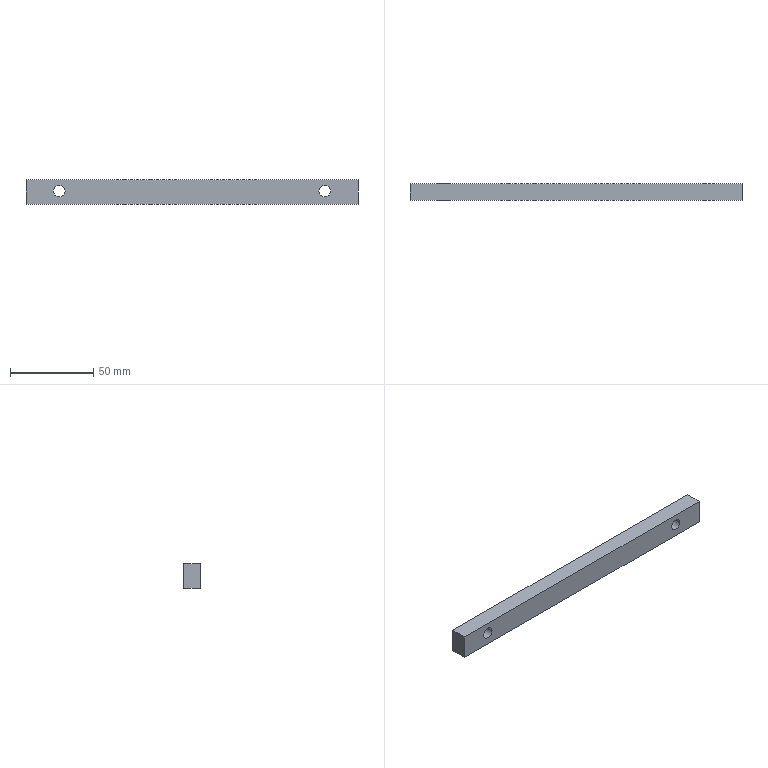Component | SolidWorks | DiscLimitPlateBasePlate-2 | 1 solid | 10 faces | box 200 x 10 x 15 mm | volume 29230 mm3 | plane 6 | cylinder 4 | commonest cylinder face diameters 7 x4
build123d program:
from build123d import *

# Parameters (mm, degrees)
SKETCH1_W      = 200
SKETCH1_H      = 15
SKETCH1_R      = 3.5
EXTRUDE1_DEPTH = 10


with BuildPart() as part:
    # Sketch1 → Extrude1 (new body)
    with BuildSketch(Plane.XY):
        with Locations((71.203, -2.922)):
            Rectangle(SKETCH1_W, SKETCH1_H)
        with Locations((-8.797, -3.422)):
            Circle(SKETCH1_R, mode=Mode.SUBTRACT)
        with Locations((151.203, -3.422)):
            Circle(SKETCH1_R, mode=Mode.SUBTRACT)
    extrude(amount=EXTRUDE1_DEPTH)


solid = part.part

# Placed as in the assembly
solid = solid.moved(Location((-235.987, 430.983, -231.751), (-90, 0, 0)))
STEP:
#1=CARTESIAN_POINT('',(-3.476,17.362,-8.989));
#2=VERTEX_POINT('',#1);
#3=CARTESIAN_POINT('',(-3.2,17.362,-8.989));
#4=VERTEX_POINT('',#3);
#5=CARTESIAN_POINT('',(-3.338,17.362,-8.989));
#6=DIRECTION('',(0.,1.,0.));
#7=DIRECTION('',(1.,0.,0.));
#8=AXIS2_PLACEMENT_3D('',#5,#6,#7);
#9=CIRCLE('',#8,0.1378);
#10=EDGE_CURVE('',#2,#4,#9,.T.);
#11=ORIENTED_EDGE('',*,*,#10,.T.);
#12=CARTESIAN_POINT('',(-3.2,16.968,-8.989));
#13=VERTEX_POINT('',#12);
#14=CARTESIAN_POINT('',(-3.2,17.362,-8.989));
#15=DIRECTION('',(0.,-1.,0.));
#16=VECTOR('',#15,39.37);
#17=LINE('',#14,#16);
#18=EDGE_CURVE('',#4,#13,#17,.T.);
#19=ORIENTED_EDGE('',*,*,#18,.T.);
#20=CARTESIAN_POINT('',(-3.476,16.968,-8.989));
#21=VERTEX_POINT('',#20);
#22=CARTESIAN_POINT('',(-3.338,16.968,-8.989));
#23=DIRECTION('',(0.,1.,0.));
#24=DIRECTION('',(1.,0.,0.));
#25=AXIS2_PLACEMENT_3D('',#22,#23,#24);
#26=CIRCLE('',#25,0.1378);
#27=EDGE_CURVE('',#21,#13,#26,.T.);
#28=ORIENTED_EDGE('',*,*,#27,.F.);
#29=CARTESIAN_POINT('',(-3.476,17.362,-8.989));
#30=DIRECTION('',(0.,-1.,0.));
#31=VECTOR('',#30,39.37);
#32=LINE('',#29,#31);
#33=EDGE_CURVE('',#2,#21,#32,.T.);
#34=ORIENTED_EDGE('',*,*,#33,.F.);
#35=EDGE_LOOP('',(#11,#19,#28,#34));
#36=FACE_OUTER_BOUND('',#35,.T.);
#37=CARTESIAN_POINT('',(-3.338,17.362,-8.989));
#38=DIRECTION('',(0.,-1.,0.));
#39=DIRECTION('',(-1.,0.,0.));
#40=AXIS2_PLACEMENT_3D('',#37,#38,#39);
#41=CYLINDRICAL_SURFACE('',#40,0.1378);
#42=ADVANCED_FACE('',(#36),#41,.F.);
#43=CARTESIAN_POINT('',(-9.775,17.362,-8.989));
#44=VERTEX_POINT('',#43);
#45=CARTESIAN_POINT('',(-9.499,17.362,-8.989));
#46=VERTEX_POINT('',#45);
#47=CARTESIAN_POINT('',(-9.637,17.362,-8.989));
#48=DIRECTION('',(0.,1.,0.));
#49=DIRECTION('',(1.,0.,0.));
#50=AXIS2_PLACEMENT_3D('',#47,#48,#49);
#51=CIRCLE('',#50,0.1378);
#52=EDGE_CURVE('',#44,#46,#51,.T.);
#53=ORIENTED_EDGE('',*,*,#52,.T.);
#54=CARTESIAN_POINT('',(-9.499,16.968,-8.989));
#55=VERTEX_POINT('',#54);
#56=CARTESIAN_POINT('',(-9.499,17.362,-8.989));
#57=DIRECTION('',(0.,-1.,0.));
#58=VECTOR('',#57,39.37);
#59=LINE('',#56,#58);
#60=EDGE_CURVE('',#46,#55,#59,.T.);
#61=ORIENTED_EDGE('',*,*,#60,.T.);
#62=CARTESIAN_POINT('',(-9.775,16.968,-8.989));
#63=VERTEX_POINT('',#62);
#64=CARTESIAN_POINT('',(-9.637,16.968,-8.989));
#65=DIRECTION('',(0.,1.,0.));
#66=DIRECTION('',(1.,0.,0.));
#67=AXIS2_PLACEMENT_3D('',#64,#65,#66);
#68=CIRCLE('',#67,0.1378);
#69=EDGE_CURVE('',#63,#55,#68,.T.);
#70=ORIENTED_EDGE('',*,*,#69,.F.);
#71=CARTESIAN_POINT('',(-9.775,17.362,-8.989));
#72=DIRECTION('',(0.,-1.,0.));
#73=VECTOR('',#72,39.37);
#74=LINE('',#71,#73);
#75=EDGE_CURVE('',#44,#63,#74,.T.);
#76=ORIENTED_EDGE('',*,*,#75,.F.);
#77=EDGE_LOOP('',(#53,#61,#70,#76));
#78=FACE_OUTER_BOUND('',#77,.T.);
#79=CARTESIAN_POINT('',(-9.637,17.362,-8.989));
#80=DIRECTION('',(0.,-1.,0.));
#81=DIRECTION('',(-1.,0.,0.));
#82=AXIS2_PLACEMENT_3D('',#79,#80,#81);
#83=CYLINDRICAL_SURFACE('',#82,0.1378);
#84=ADVANCED_FACE('',(#78),#83,.F.);
#85=ORIENTED_EDGE('',*,*,#52,.F.);
#86=CARTESIAN_POINT('',(-9.637,17.362,-8.989));
#87=DIRECTION('',(0.,1.,0.));
#88=DIRECTION('',(1.,0.,0.));
#89=AXIS2_PLACEMENT_3D('',#86,#87,#88);
#90=CIRCLE('',#89,0.1378);
#91=EDGE_CURVE('',#46,#44,#90,.T.);
#92=ORIENTED_EDGE('',*,*,#91,.F.);
#93=EDGE_LOOP('',(#85,#92));
#94=FACE_BOUND('',#93,.T.);
#95=CARTESIAN_POINT('',(-10.425,17.362,-9.304));
#96=VERTEX_POINT('',#95);
#97=CARTESIAN_POINT('',(-10.425,17.362,-8.714));
#98=VERTEX_POINT('',#97);
#99=CARTESIAN_POINT('',(-10.425,17.362,-9.304));
#100=DIRECTION('',(0.,0.,1.));
#101=VECTOR('',#100,39.37);
#102=LINE('',#99,#101);
#103=EDGE_CURVE('',#96,#98,#102,.T.);
#104=ORIENTED_EDGE('',*,*,#103,.T.);
#105=CARTESIAN_POINT('',(-2.551,17.362,-8.714));
#106=VERTEX_POINT('',#105);
#107=CARTESIAN_POINT('',(-10.425,17.362,-8.714));
#108=DIRECTION('',(1.,0.,0.));
#109=VECTOR('',#108,39.37);
#110=LINE('',#107,#109);
#111=EDGE_CURVE('',#98,#106,#110,.T.);
#112=ORIENTED_EDGE('',*,*,#111,.T.);
#113=CARTESIAN_POINT('',(-2.551,17.362,-9.304));
#114=VERTEX_POINT('',#113);
#115=CARTESIAN_POINT('',(-2.551,17.362,-9.304));
#116=DIRECTION('',(0.,0.,-1.));
#117=VECTOR('',#116,39.37);
#118=LINE('',#115,#117);
#119=EDGE_CURVE('',#106,#114,#118,.T.);
#120=ORIENTED_EDGE('',*,*,#119,.T.);
#121=CARTESIAN_POINT('',(-10.425,17.362,-9.304));
#122=DIRECTION('',(-1.,0.,0.));
#123=VECTOR('',#122,39.37);
#124=LINE('',#121,#123);
#125=EDGE_CURVE('',#114,#96,#124,.T.);
#126=ORIENTED_EDGE('',*,*,#125,.T.);
#127=EDGE_LOOP('',(#104,#112,#120,#126));
#128=FACE_OUTER_BOUND('',#127,.T.);
#129=ORIENTED_EDGE('',*,*,#10,.F.);
#130=CARTESIAN_POINT('',(-3.338,17.362,-8.989));
#131=DIRECTION('',(0.,1.,0.));
#132=DIRECTION('',(1.,0.,0.));
#133=AXIS2_PLACEMENT_3D('',#130,#131,#132);
#134=CIRCLE('',#133,0.1378);
#135=EDGE_CURVE('',#4,#2,#134,.T.);
#136=ORIENTED_EDGE('',*,*,#135,.F.);
#137=EDGE_LOOP('',(#129,#136));
#138=FACE_BOUND('',#137,.T.);
#139=CARTESIAN_POINT('',(-10.425,17.362,-8.714));
#140=DIRECTION('',(0.,1.,0.));
#141=DIRECTION('',(1.,0.,0.));
#142=AXIS2_PLACEMENT_3D('',#139,#140,#141);
#143=PLANE('',#142);
#144=ADVANCED_FACE('',(#94,#128,#138),#143,.T.);
#145=CARTESIAN_POINT('',(-10.425,16.968,-9.304));
#146=VERTEX_POINT('',#145);
#147=CARTESIAN_POINT('',(-10.425,16.968,-8.714));
#148=VERTEX_POINT('',#147);
#149=CARTESIAN_POINT('',(-10.425,16.968,-9.304));
#150=DIRECTION('',(0.,0.,1.));
#151=VECTOR('',#150,39.37);
#152=LINE('',#149,#151);
#153=EDGE_CURVE('',#146,#148,#152,.T.);
#154=ORIENTED_EDGE('',*,*,#153,.F.);
#155=CARTESIAN_POINT('',(-2.551,16.968,-9.304));
#156=VERTEX_POINT('',#155);
#157=CARTESIAN_POINT('',(-10.425,16.968,-9.304));
#158=DIRECTION('',(-1.,0.,0.));
#159=VECTOR('',#158,39.37);
#160=LINE('',#157,#159);
#161=EDGE_CURVE('',#156,#146,#160,.T.);
#162=ORIENTED_EDGE('',*,*,#161,.F.);
#163=CARTESIAN_POINT('',(-2.551,16.968,-8.714));
#164=VERTEX_POINT('',#163);
#165=CARTESIAN_POINT('',(-2.551,16.968,-9.304));
#166=DIRECTION('',(0.,0.,-1.));
#167=VECTOR('',#166,39.37);
#168=LINE('',#165,#167);
#169=EDGE_CURVE('',#164,#156,#168,.T.);
#170=ORIENTED_EDGE('',*,*,#169,.F.);
#171=CARTESIAN_POINT('',(-10.425,16.968,-8.714));
#172=DIRECTION('',(1.,0.,0.));
#173=VECTOR('',#172,39.37);
#174=LINE('',#171,#173);
#175=EDGE_CURVE('',#148,#164,#174,.T.);
#176=ORIENTED_EDGE('',*,*,#175,.F.);
#177=EDGE_LOOP('',(#154,#162,#170,#176));
#178=FACE_OUTER_BOUND('',#177,.T.);
#179=ORIENTED_EDGE('',*,*,#69,.T.);
#180=CARTESIAN_POINT('',(-9.637,16.968,-8.989));
#181=DIRECTION('',(0.,1.,0.));
#182=DIRECTION('',(1.,0.,0.));
#183=AXIS2_PLACEMENT_3D('',#180,#181,#182);
#184=CIRCLE('',#183,0.1378);
#185=EDGE_CURVE('',#55,#63,#184,.T.);
#186=ORIENTED_EDGE('',*,*,#185,.T.);
#187=EDGE_LOOP('',(#179,#186));
#188=FACE_BOUND('',#187,.T.);
#189=ORIENTED_EDGE('',*,*,#27,.T.);
#190=CARTESIAN_POINT('',(-3.338,16.968,-8.989));
#191=DIRECTION('',(0.,1.,0.));
#192=DIRECTION('',(1.,0.,0.));
#193=AXIS2_PLACEMENT_3D('',#190,#191,#192);
#194=CIRCLE('',#193,0.1378);
#195=EDGE_CURVE('',#13,#21,#194,.T.);
#196=ORIENTED_EDGE('',*,*,#195,.T.);
#197=EDGE_LOOP('',(#189,#196));
#198=FACE_BOUND('',#197,.T.);
#199=CARTESIAN_POINT('',(-10.425,16.968,-8.714));
#200=DIRECTION('',(0.,1.,0.));
#201=DIRECTION('',(1.,0.,0.));
#202=AXIS2_PLACEMENT_3D('',#199,#200,#201);
#203=PLANE('',#202);
#204=ADVANCED_FACE('',(#178,#188,#198),#203,.F.);
#205=ORIENTED_EDGE('',*,*,#153,.T.);
#206=CARTESIAN_POINT('',(-10.425,17.362,-8.714));
#207=DIRECTION('',(0.,-1.,0.));
#208=VECTOR('',#207,39.37);
#209=LINE('',#206,#208);
#210=EDGE_CURVE('',#98,#148,#209,.T.);
#211=ORIENTED_EDGE('',*,*,#210,.F.);
#212=ORIENTED_EDGE('',*,*,#103,.F.);
#213=CARTESIAN_POINT('',(-10.425,17.362,-9.304));
#214=DIRECTION('',(0.,-1.,0.));
#215=VECTOR('',#214,39.37);
#216=LINE('',#213,#215);
#217=EDGE_CURVE('',#96,#146,#216,.T.);
#218=ORIENTED_EDGE('',*,*,#217,.T.);
#219=EDGE_LOOP('',(#205,#211,#212,#218));
#220=FACE_OUTER_BOUND('',#219,.T.);
#221=CARTESIAN_POINT('',(-10.425,17.362,-9.304));
#222=DIRECTION('',(1.,0.,-0.));
#223=DIRECTION('',(-0.,0.,-1.));
#224=AXIS2_PLACEMENT_3D('',#221,#222,#223);
#225=PLANE('',#224);
#226=ADVANCED_FACE('',(#220),#225,.F.);
#227=ORIENTED_EDGE('',*,*,#175,.T.);
#228=CARTESIAN_POINT('',(-2.551,17.362,-8.714));
#229=DIRECTION('',(0.,-1.,0.));
#230=VECTOR('',#229,39.37);
#231=LINE('',#228,#230);
#232=EDGE_CURVE('',#106,#164,#231,.T.);
#233=ORIENTED_EDGE('',*,*,#232,.F.);
#234=ORIENTED_EDGE('',*,*,#111,.F.);
#235=ORIENTED_EDGE('',*,*,#210,.T.);
#236=EDGE_LOOP('',(#227,#233,#234,#235));
#237=FACE_OUTER_BOUND('',#236,.T.);
#238=CARTESIAN_POINT('',(-10.425,17.362,-8.714));
#239=DIRECTION('',(0.,0.,-1.));
#240=DIRECTION('',(0.,1.,0.));
#241=AXIS2_PLACEMENT_3D('',#238,#239,#240);
#242=PLANE('',#241);
#243=ADVANCED_FACE('',(#237),#242,.F.);
#244=ORIENTED_EDGE('',*,*,#169,.T.);
#245=CARTESIAN_POINT('',(-2.551,17.362,-9.304));
#246=DIRECTION('',(0.,-1.,0.));
#247=VECTOR('',#246,39.37);
#248=LINE('',#245,#247);
#249=EDGE_CURVE('',#114,#156,#248,.T.);
#250=ORIENTED_EDGE('',*,*,#249,.F.);
#251=ORIENTED_EDGE('',*,*,#119,.F.);
#252=ORIENTED_EDGE('',*,*,#232,.T.);
#253=EDGE_LOOP('',(#244,#250,#251,#252));
#254=FACE_OUTER_BOUND('',#253,.T.);
#255=CARTESIAN_POINT('',(-2.551,17.362,-9.304));
#256=DIRECTION('',(-1.,0.,0.));
#257=DIRECTION('',(0.,1.,0.));
#258=AXIS2_PLACEMENT_3D('',#255,#256,#257);
#259=PLANE('',#258);
#260=ADVANCED_FACE('',(#254),#259,.F.);
#261=ORIENTED_EDGE('',*,*,#161,.T.);
#262=ORIENTED_EDGE('',*,*,#217,.F.);
#263=ORIENTED_EDGE('',*,*,#125,.F.);
#264=ORIENTED_EDGE('',*,*,#249,.T.);
#265=EDGE_LOOP('',(#261,#262,#263,#264));
#266=FACE_OUTER_BOUND('',#265,.T.);
#267=CARTESIAN_POINT('',(-10.425,17.362,-9.304));
#268=DIRECTION('',(0.,0.,1.));
#269=DIRECTION('',(0.,-1.,0.));
#270=AXIS2_PLACEMENT_3D('',#267,#268,#269);
#271=PLANE('',#270);
#272=ADVANCED_FACE('',(#266),#271,.F.);
#273=ORIENTED_EDGE('',*,*,#60,.F.);
#274=ORIENTED_EDGE('',*,*,#91,.T.);
#275=ORIENTED_EDGE('',*,*,#75,.T.);
#276=ORIENTED_EDGE('',*,*,#185,.F.);
#277=EDGE_LOOP('',(#273,#274,#275,#276));
#278=FACE_OUTER_BOUND('',#277,.T.);
#279=CARTESIAN_POINT('',(-9.637,17.362,-8.989));
#280=DIRECTION('',(0.,-1.,0.));
#281=DIRECTION('',(-1.,0.,0.));
#282=AXIS2_PLACEMENT_3D('',#279,#280,#281);
#283=CYLINDRICAL_SURFACE('',#282,0.1378);
#284=ADVANCED_FACE('',(#278),#283,.F.);
#285=ORIENTED_EDGE('',*,*,#18,.F.);
#286=ORIENTED_EDGE('',*,*,#135,.T.);
#287=ORIENTED_EDGE('',*,*,#33,.T.);
#288=ORIENTED_EDGE('',*,*,#195,.F.);
#289=EDGE_LOOP('',(#285,#286,#287,#288));
#290=FACE_OUTER_BOUND('',#289,.T.);
#291=CARTESIAN_POINT('',(-3.338,17.362,-8.989));
#292=DIRECTION('',(0.,-1.,0.));
#293=DIRECTION('',(-1.,0.,0.));
#294=AXIS2_PLACEMENT_3D('',#291,#292,#293);
#295=CYLINDRICAL_SURFACE('',#294,0.1378);
#296=ADVANCED_FACE('',(#290),#295,.F.);
#297=CLOSED_SHELL('',(#42,#84,#144,#204,#226,#243,#260,#272,#284,#296));
#298=MANIFOLD_SOLID_BREP('',#297);
#299=CARTESIAN_POINT('',(0.,0.,0.));
#300=DIRECTION('',(0.,0.,1.));
#301=DIRECTION('',(1.,0.,0.));
#302=AXIS2_PLACEMENT_3D('',#299,#300,#301);
#303=(LENGTH_UNIT()NAMED_UNIT(*)SI_UNIT($,.METRE.));
#304=LENGTH_MEASURE_WITH_UNIT(LENGTH_MEASURE(0.0254),#303);
#305=DIMENSIONAL_EXPONENTS(1.,0.,0.,0.,0.,0.,0.);
#306=(CONVERSION_BASED_UNIT('',#304)LENGTH_UNIT()NAMED_UNIT(#305));
#307=UNCERTAINTY_MEASURE_WITH_UNIT(LENGTH_MEASURE(0.00001),#306,'','');
#308=(NAMED_UNIT(*)PLANE_ANGLE_UNIT()SI_UNIT($,.RADIAN.));
#309=(NAMED_UNIT(*)SI_UNIT($,.STERADIAN.)SOLID_ANGLE_UNIT());
#310=(GEOMETRIC_REPRESENTATION_CONTEXT(3)GLOBAL_UNCERTAINTY_ASSIGNED_CONTEXT((#307))GLOBAL_UNIT_ASSIGNED_CONTEXT((#306,#308,#309))REPRESENTATION_CONTEXT('',''));
#311=ADVANCED_BREP_SHAPE_REPRESENTATION('',(#298,#302),#310);
#312=COLOUR_RGB('',0.7922,0.8196,0.9333);
#313=FILL_AREA_STYLE_COLOUR('',#312);
#314=FILL_AREA_STYLE('',(#313));
#315=SURFACE_STYLE_FILL_AREA(#314);
#316=SURFACE_SIDE_STYLE('',(#315));
#317=SURFACE_STYLE_USAGE(.BOTH.,#316);
#318=PRESENTATION_STYLE_ASSIGNMENT((#317));
#319=STYLED_ITEM('',(#318),#298);
#320=PRESENTATION_LAYER_ASSIGNMENT('','',(#319));
#321=(LENGTH_UNIT()NAMED_UNIT(*)SI_UNIT($,.METRE.));
#322=LENGTH_MEASURE_WITH_UNIT(LENGTH_MEASURE(0.0254),#321);
#323=DIMENSIONAL_EXPONENTS(1.,0.,0.,0.,0.,0.,0.);
#324=(CONVERSION_BASED_UNIT('',#322)LENGTH_UNIT()NAMED_UNIT(#323));
#325=UNCERTAINTY_MEASURE_WITH_UNIT(LENGTH_MEASURE(0.00001),#324,'','');
#326=(NAMED_UNIT(*)PLANE_ANGLE_UNIT()SI_UNIT($,.RADIAN.));
#327=(NAMED_UNIT(*)SI_UNIT($,.STERADIAN.)SOLID_ANGLE_UNIT());
#328=(GEOMETRIC_REPRESENTATION_CONTEXT(3)GLOBAL_UNCERTAINTY_ASSIGNED_CONTEXT((#325))GLOBAL_UNIT_ASSIGNED_CONTEXT((#324,#326,#327))REPRESENTATION_CONTEXT('',''));
#329=MECHANICAL_DESIGN_GEOMETRIC_PRESENTATION_REPRESENTATION('',(#319),#328);